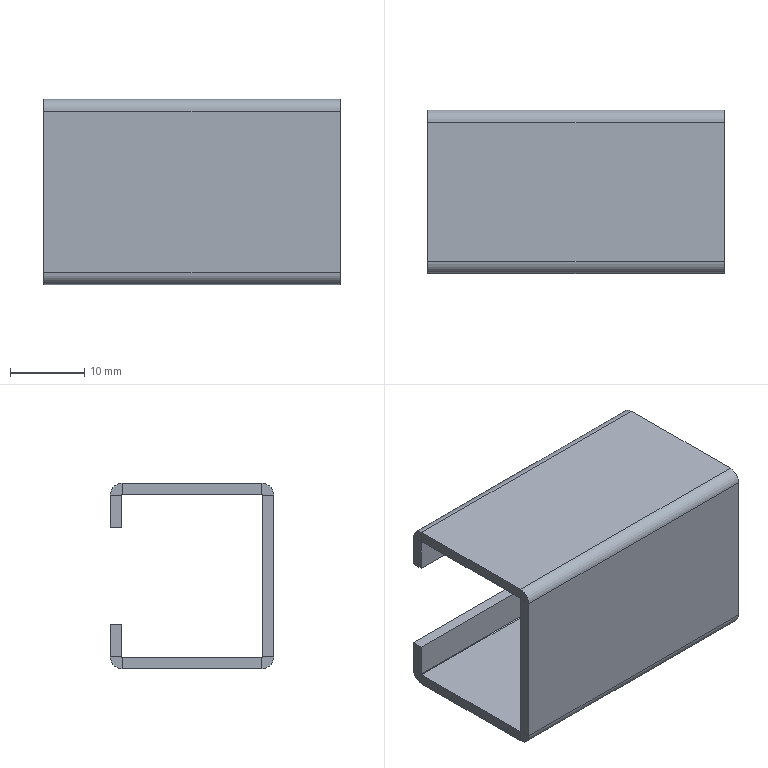Component | SolidWorks | FrontDoorAssembly-1_FrontDoorWelding-1_DoorLockBarGuideSeatPG50-02-106-1 | 1 solid | 38 faces | box 40 x 22 x 25 mm | volume 4412 mm3 | plane 30 | cylinder 8 | commonest cylinder face diameters 3.2 x4 0.2 x4 | material AISI 1045 Steel, cold drawn
STEP:
#1=CARTESIAN_POINT('',(-39.122,-10.291,15.187));
#2=VERTEX_POINT('',#1);
#3=CARTESIAN_POINT('',(-39.122,-10.291,15.246));
#4=VERTEX_POINT('',#3);
#5=CARTESIAN_POINT('',(-39.122,-10.291,15.187));
#6=DIRECTION('',(0.,0.,1.));
#7=VECTOR('',#6,39.37);
#8=LINE('',#5,#7);
#9=EDGE_CURVE('',#2,#4,#8,.T.);
#10=ORIENTED_EDGE('',*,*,#9,.F.);
#11=CARTESIAN_POINT('',(-39.122,-11.031,15.187));
#12=VERTEX_POINT('',#11);
#13=CARTESIAN_POINT('',(-39.122,-11.035,15.187));
#14=DIRECTION('',(0.,-1.,-0.));
#15=VECTOR('',#14,39.37);
#16=LINE('',#13,#15);
#17=EDGE_CURVE('',#2,#12,#16,.T.);
#18=ORIENTED_EDGE('',*,*,#17,.T.);
#19=CARTESIAN_POINT('',(-39.122,-11.031,15.246));
#20=VERTEX_POINT('',#19);
#21=CARTESIAN_POINT('',(-39.122,-11.031,15.246));
#22=DIRECTION('',(0.,-0.,1.));
#23=VECTOR('',#22,39.37);
#24=LINE('',#21,#23);
#25=EDGE_CURVE('',#12,#20,#24,.T.);
#26=ORIENTED_EDGE('',*,*,#25,.T.);
#27=CARTESIAN_POINT('',(-39.122,-11.035,15.246));
#28=DIRECTION('',(0.,-1.,-0.));
#29=VECTOR('',#28,39.37);
#30=LINE('',#27,#29);
#31=EDGE_CURVE('',#4,#20,#30,.T.);
#32=ORIENTED_EDGE('',*,*,#31,.F.);
#33=EDGE_LOOP('',(#10,#18,#26,#32));
#34=FACE_OUTER_BOUND('',#33,.T.);
#35=CARTESIAN_POINT('',(-39.122,-11.035,15.246));
#36=DIRECTION('',(1.,0.,-0.));
#37=DIRECTION('',(-0.,-0.,-1.));
#38=AXIS2_PLACEMENT_3D('',#35,#36,#37);
#39=PLANE('',#38);
#40=ADVANCED_FACE('',(#34),#39,.F.);
#41=CARTESIAN_POINT('',(-37.547,-10.291,15.187));
#42=VERTEX_POINT('',#41);
#43=CARTESIAN_POINT('',(-37.547,-10.291,15.246));
#44=VERTEX_POINT('',#43);
#45=CARTESIAN_POINT('',(-37.547,-10.291,15.187));
#46=DIRECTION('',(0.,0.,1.));
#47=VECTOR('',#46,39.37);
#48=LINE('',#45,#47);
#49=EDGE_CURVE('',#42,#44,#48,.T.);
#50=ORIENTED_EDGE('',*,*,#49,.T.);
#51=CARTESIAN_POINT('',(-37.547,-11.031,15.246));
#52=VERTEX_POINT('',#51);
#53=CARTESIAN_POINT('',(-37.547,-11.035,15.246));
#54=DIRECTION('',(-0.,1.,0.));
#55=VECTOR('',#54,39.37);
#56=LINE('',#53,#55);
#57=EDGE_CURVE('',#52,#44,#56,.T.);
#58=ORIENTED_EDGE('',*,*,#57,.F.);
#59=CARTESIAN_POINT('',(-37.547,-11.031,15.187));
#60=VERTEX_POINT('',#59);
#61=CARTESIAN_POINT('',(-37.547,-11.031,15.187));
#62=DIRECTION('',(0.,-0.,1.));
#63=VECTOR('',#62,39.37);
#64=LINE('',#61,#63);
#65=EDGE_CURVE('',#60,#52,#64,.T.);
#66=ORIENTED_EDGE('',*,*,#65,.F.);
#67=CARTESIAN_POINT('',(-37.547,-10.228,15.187));
#68=DIRECTION('',(-0.,1.,0.));
#69=VECTOR('',#68,39.37);
#70=LINE('',#67,#69);
#71=EDGE_CURVE('',#60,#42,#70,.T.);
#72=ORIENTED_EDGE('',*,*,#71,.T.);
#73=EDGE_LOOP('',(#50,#58,#66,#72));
#74=FACE_OUTER_BOUND('',#73,.T.);
#75=CARTESIAN_POINT('',(-37.547,-10.228,15.246));
#76=DIRECTION('',(-1.,-0.,0.));
#77=DIRECTION('',(0.,0.,1.));
#78=AXIS2_PLACEMENT_3D('',#75,#76,#77);
#79=PLANE('',#78);
#80=ADVANCED_FACE('',(#74),#79,.F.);
#81=CARTESIAN_POINT('',(-37.547,-10.291,15.246));
#82=DIRECTION('',(-1.,-0.,0.));
#83=VECTOR('',#82,39.37);
#84=LINE('',#81,#83);
#85=EDGE_CURVE('',#44,#4,#84,.T.);
#86=ORIENTED_EDGE('',*,*,#85,.T.);
#87=ORIENTED_EDGE('',*,*,#31,.T.);
#88=CARTESIAN_POINT('',(-39.122,-11.031,15.246));
#89=DIRECTION('',(-1.,-0.,0.));
#90=VECTOR('',#89,39.37);
#91=LINE('',#88,#90);
#92=EDGE_CURVE('',#52,#20,#91,.T.);
#93=ORIENTED_EDGE('',*,*,#92,.F.);
#94=ORIENTED_EDGE('',*,*,#57,.T.);
#95=EDGE_LOOP('',(#86,#87,#93,#94));
#96=FACE_OUTER_BOUND('',#95,.T.);
#97=CARTESIAN_POINT('',(-38.334,-11.035,15.246));
#98=DIRECTION('',(-0.,0.,-1.));
#99=DIRECTION('',(-0.,1.,0.));
#100=AXIS2_PLACEMENT_3D('',#97,#98,#99);
#101=PLANE('',#100);
#102=ADVANCED_FACE('',(#96),#101,.F.);
#103=ORIENTED_EDGE('',*,*,#17,.F.);
#104=CARTESIAN_POINT('',(-37.547,-10.291,15.187));
#105=DIRECTION('',(-1.,-0.,0.));
#106=VECTOR('',#105,39.37);
#107=LINE('',#104,#106);
#108=EDGE_CURVE('',#42,#2,#107,.T.);
#109=ORIENTED_EDGE('',*,*,#108,.F.);
#110=ORIENTED_EDGE('',*,*,#71,.F.);
#111=CARTESIAN_POINT('',(-39.122,-11.031,15.187));
#112=DIRECTION('',(1.,0.,-0.));
#113=VECTOR('',#112,39.37);
#114=LINE('',#111,#113);
#115=EDGE_CURVE('',#12,#60,#114,.T.);
#116=ORIENTED_EDGE('',*,*,#115,.F.);
#117=EDGE_LOOP('',(#103,#109,#110,#116));
#118=FACE_OUTER_BOUND('',#117,.T.);
#119=CARTESIAN_POINT('',(-38.334,-11.035,15.187));
#120=DIRECTION('',(-0.,0.,-1.));
#121=DIRECTION('',(-0.,1.,0.));
#122=AXIS2_PLACEMENT_3D('',#119,#120,#121);
#123=PLANE('',#122);
#124=ADVANCED_FACE('',(#118),#123,.T.);
#125=CARTESIAN_POINT('',(-37.547,-10.291,14.321));
#126=VERTEX_POINT('',#125);
#127=CARTESIAN_POINT('',(-37.547,-10.291,14.262));
#128=VERTEX_POINT('',#127);
#129=CARTESIAN_POINT('',(-37.547,-10.291,14.321));
#130=DIRECTION('',(-0.,-0.,-1.));
#131=VECTOR('',#130,39.37);
#132=LINE('',#129,#131);
#133=EDGE_CURVE('',#126,#128,#132,.T.);
#134=ORIENTED_EDGE('',*,*,#133,.F.);
#135=CARTESIAN_POINT('',(-37.547,-11.031,14.321));
#136=VERTEX_POINT('',#135);
#137=CARTESIAN_POINT('',(-37.547,-11.035,14.321));
#138=DIRECTION('',(0.,-1.,0.));
#139=VECTOR('',#138,39.37);
#140=LINE('',#137,#139);
#141=EDGE_CURVE('',#126,#136,#140,.T.);
#142=ORIENTED_EDGE('',*,*,#141,.T.);
#143=CARTESIAN_POINT('',(-37.547,-11.031,14.262));
#144=VERTEX_POINT('',#143);
#145=CARTESIAN_POINT('',(-37.547,-11.031,14.262));
#146=DIRECTION('',(-0.,-0.,-1.));
#147=VECTOR('',#146,39.37);
#148=LINE('',#145,#147);
#149=EDGE_CURVE('',#136,#144,#148,.T.);
#150=ORIENTED_EDGE('',*,*,#149,.T.);
#151=CARTESIAN_POINT('',(-37.547,-11.035,14.262));
#152=DIRECTION('',(0.,-1.,0.));
#153=VECTOR('',#152,39.37);
#154=LINE('',#151,#153);
#155=EDGE_CURVE('',#128,#144,#154,.T.);
#156=ORIENTED_EDGE('',*,*,#155,.F.);
#157=EDGE_LOOP('',(#134,#142,#150,#156));
#158=FACE_OUTER_BOUND('',#157,.T.);
#159=CARTESIAN_POINT('',(-37.547,-11.035,14.262));
#160=DIRECTION('',(-1.,-0.,0.));
#161=DIRECTION('',(-0.,1.,0.));
#162=AXIS2_PLACEMENT_3D('',#159,#160,#161);
#163=PLANE('',#162);
#164=ADVANCED_FACE('',(#158),#163,.F.);
#165=CARTESIAN_POINT('',(-39.122,-10.291,14.321));
#166=VERTEX_POINT('',#165);
#167=CARTESIAN_POINT('',(-39.122,-10.291,14.262));
#168=VERTEX_POINT('',#167);
#169=CARTESIAN_POINT('',(-39.122,-10.291,14.321));
#170=DIRECTION('',(-0.,-0.,-1.));
#171=VECTOR('',#170,39.37);
#172=LINE('',#169,#171);
#173=EDGE_CURVE('',#166,#168,#172,.T.);
#174=ORIENTED_EDGE('',*,*,#173,.T.);
#175=CARTESIAN_POINT('',(-39.122,-11.031,14.262));
#176=VERTEX_POINT('',#175);
#177=CARTESIAN_POINT('',(-39.122,-11.035,14.262));
#178=DIRECTION('',(-0.,1.,-0.));
#179=VECTOR('',#178,39.37);
#180=LINE('',#177,#179);
#181=EDGE_CURVE('',#176,#168,#180,.T.);
#182=ORIENTED_EDGE('',*,*,#181,.F.);
#183=CARTESIAN_POINT('',(-39.122,-11.031,14.321));
#184=VERTEX_POINT('',#183);
#185=CARTESIAN_POINT('',(-39.122,-11.031,14.321));
#186=DIRECTION('',(-0.,-0.,-1.));
#187=VECTOR('',#186,39.37);
#188=LINE('',#185,#187);
#189=EDGE_CURVE('',#184,#176,#188,.T.);
#190=ORIENTED_EDGE('',*,*,#189,.F.);
#191=CARTESIAN_POINT('',(-39.122,-10.228,14.321));
#192=DIRECTION('',(-0.,1.,-0.));
#193=VECTOR('',#192,39.37);
#194=LINE('',#191,#193);
#195=EDGE_CURVE('',#184,#166,#194,.T.);
#196=ORIENTED_EDGE('',*,*,#195,.T.);
#197=EDGE_LOOP('',(#174,#182,#190,#196));
#198=FACE_OUTER_BOUND('',#197,.T.);
#199=CARTESIAN_POINT('',(-39.122,-10.228,14.262));
#200=DIRECTION('',(1.,0.,-0.));
#201=DIRECTION('',(0.,-1.,-0.));
#202=AXIS2_PLACEMENT_3D('',#199,#200,#201);
#203=PLANE('',#202);
#204=ADVANCED_FACE('',(#198),#203,.F.);
#205=CARTESIAN_POINT('',(-39.122,-10.291,14.262));
#206=DIRECTION('',(1.,0.,-0.));
#207=VECTOR('',#206,39.37);
#208=LINE('',#205,#207);
#209=EDGE_CURVE('',#168,#128,#208,.T.);
#210=ORIENTED_EDGE('',*,*,#209,.T.);
#211=ORIENTED_EDGE('',*,*,#155,.T.);
#212=CARTESIAN_POINT('',(-37.547,-11.031,14.262));
#213=DIRECTION('',(1.,0.,-0.));
#214=VECTOR('',#213,39.37);
#215=LINE('',#212,#214);
#216=EDGE_CURVE('',#176,#144,#215,.T.);
#217=ORIENTED_EDGE('',*,*,#216,.F.);
#218=ORIENTED_EDGE('',*,*,#181,.T.);
#219=EDGE_LOOP('',(#210,#211,#217,#218));
#220=FACE_OUTER_BOUND('',#219,.T.);
#221=CARTESIAN_POINT('',(-38.334,-11.035,14.262));
#222=DIRECTION('',(0.,0.,1.));
#223=DIRECTION('',(0.,-1.,0.));
#224=AXIS2_PLACEMENT_3D('',#221,#222,#223);
#225=PLANE('',#224);
#226=ADVANCED_FACE('',(#220),#225,.F.);
#227=ORIENTED_EDGE('',*,*,#141,.F.);
#228=CARTESIAN_POINT('',(-39.122,-10.291,14.321));
#229=DIRECTION('',(1.,0.,-0.));
#230=VECTOR('',#229,39.37);
#231=LINE('',#228,#230);
#232=EDGE_CURVE('',#166,#126,#231,.T.);
#233=ORIENTED_EDGE('',*,*,#232,.F.);
#234=ORIENTED_EDGE('',*,*,#195,.F.);
#235=CARTESIAN_POINT('',(-37.547,-11.031,14.321));
#236=DIRECTION('',(-1.,-0.,0.));
#237=VECTOR('',#236,39.37);
#238=LINE('',#235,#237);
#239=EDGE_CURVE('',#136,#184,#238,.T.);
#240=ORIENTED_EDGE('',*,*,#239,.F.);
#241=EDGE_LOOP('',(#227,#233,#234,#240));
#242=FACE_OUTER_BOUND('',#241,.T.);
#243=CARTESIAN_POINT('',(-38.334,-11.035,14.321));
#244=DIRECTION('',(0.,0.,1.));
#245=DIRECTION('',(0.,-1.,0.));
#246=AXIS2_PLACEMENT_3D('',#243,#244,#245);
#247=PLANE('',#246);
#248=ADVANCED_FACE('',(#242),#247,.T.);
#249=CARTESIAN_POINT('',(-37.547,-11.094,15.183));
#250=VERTEX_POINT('',#249);
#251=CARTESIAN_POINT('',(-37.547,-11.094,14.325));
#252=VERTEX_POINT('',#251);
#253=CARTESIAN_POINT('',(-37.547,-11.094,14.262));
#254=DIRECTION('',(-0.,-0.,-1.));
#255=VECTOR('',#254,39.37);
#256=LINE('',#253,#255);
#257=EDGE_CURVE('',#250,#252,#256,.T.);
#258=ORIENTED_EDGE('',*,*,#257,.F.);
#259=CARTESIAN_POINT('',(-39.122,-11.094,15.183));
#260=VERTEX_POINT('',#259);
#261=CARTESIAN_POINT('',(-37.547,-11.094,15.183));
#262=DIRECTION('',(-1.,-0.,0.));
#263=VECTOR('',#262,39.37);
#264=LINE('',#261,#263);
#265=EDGE_CURVE('',#250,#260,#264,.T.);
#266=ORIENTED_EDGE('',*,*,#265,.T.);
#267=CARTESIAN_POINT('',(-39.122,-11.094,14.325));
#268=VERTEX_POINT('',#267);
#269=CARTESIAN_POINT('',(-39.122,-11.094,14.262));
#270=DIRECTION('',(0.,0.,1.));
#271=VECTOR('',#270,39.37);
#272=LINE('',#269,#271);
#273=EDGE_CURVE('',#268,#260,#272,.T.);
#274=ORIENTED_EDGE('',*,*,#273,.F.);
#275=CARTESIAN_POINT('',(-39.122,-11.094,14.325));
#276=DIRECTION('',(1.,0.,-0.));
#277=VECTOR('',#276,39.37);
#278=LINE('',#275,#277);
#279=EDGE_CURVE('',#268,#252,#278,.T.);
#280=ORIENTED_EDGE('',*,*,#279,.T.);
#281=EDGE_LOOP('',(#258,#266,#274,#280));
#282=FACE_OUTER_BOUND('',#281,.T.);
#283=CARTESIAN_POINT('',(-38.334,-11.094,14.754));
#284=DIRECTION('',(0.,-1.,-0.));
#285=DIRECTION('',(-1.,-0.,0.));
#286=AXIS2_PLACEMENT_3D('',#283,#284,#285);
#287=PLANE('',#286);
#288=ADVANCED_FACE('',(#282),#287,.T.);
#289=CARTESIAN_POINT('',(-37.547,-11.035,15.183));
#290=VERTEX_POINT('',#289);
#291=CARTESIAN_POINT('',(-39.122,-11.035,15.183));
#292=VERTEX_POINT('',#291);
#293=CARTESIAN_POINT('',(-37.547,-11.035,15.183));
#294=DIRECTION('',(-1.,-0.,0.));
#295=VECTOR('',#294,39.37);
#296=LINE('',#293,#295);
#297=EDGE_CURVE('',#290,#292,#296,.T.);
#298=ORIENTED_EDGE('',*,*,#297,.F.);
#299=CARTESIAN_POINT('',(-37.547,-11.035,14.325));
#300=VERTEX_POINT('',#299);
#301=CARTESIAN_POINT('',(-37.547,-11.035,14.262));
#302=DIRECTION('',(-0.,-0.,-1.));
#303=VECTOR('',#302,39.37);
#304=LINE('',#301,#303);
#305=EDGE_CURVE('',#290,#300,#304,.T.);
#306=ORIENTED_EDGE('',*,*,#305,.T.);
#307=CARTESIAN_POINT('',(-39.122,-11.035,14.325));
#308=VERTEX_POINT('',#307);
#309=CARTESIAN_POINT('',(-39.122,-11.035,14.325));
#310=DIRECTION('',(1.,0.,-0.));
#311=VECTOR('',#310,39.37);
#312=LINE('',#309,#311);
#313=EDGE_CURVE('',#308,#300,#312,.T.);
#314=ORIENTED_EDGE('',*,*,#313,.F.);
#315=CARTESIAN_POINT('',(-39.122,-11.035,14.262));
#316=DIRECTION('',(0.,0.,1.));
#317=VECTOR('',#316,39.37);
#318=LINE('',#315,#317);
#319=EDGE_CURVE('',#308,#292,#318,.T.);
#320=ORIENTED_EDGE('',*,*,#319,.T.);
#321=EDGE_LOOP('',(#298,#306,#314,#320));
#322=FACE_OUTER_BOUND('',#321,.T.);
#323=CARTESIAN_POINT('',(-38.334,-11.035,14.754));
#324=DIRECTION('',(0.,-1.,-0.));
#325=DIRECTION('',(-1.,-0.,0.));
#326=AXIS2_PLACEMENT_3D('',#323,#324,#325);
#327=PLANE('',#326);
#328=ADVANCED_FACE('',(#322),#327,.F.);
#329=ORIENTED_EDGE('',*,*,#305,.F.);
#330=CARTESIAN_POINT('',(-37.547,-11.035,15.183));
#331=DIRECTION('',(0.,-1.,-0.));
#332=VECTOR('',#331,39.37);
#333=LINE('',#330,#332);
#334=EDGE_CURVE('',#290,#250,#333,.T.);
#335=ORIENTED_EDGE('',*,*,#334,.T.);
#336=ORIENTED_EDGE('',*,*,#257,.T.);
#337=CARTESIAN_POINT('',(-37.547,-11.035,14.325));
#338=DIRECTION('',(0.,-1.,0.));
#339=VECTOR('',#338,39.37);
#340=LINE('',#337,#339);
#341=EDGE_CURVE('',#300,#252,#340,.T.);
#342=ORIENTED_EDGE('',*,*,#341,.F.);
#343=EDGE_LOOP('',(#329,#335,#336,#342));
#344=FACE_OUTER_BOUND('',#343,.T.);
#345=CARTESIAN_POINT('',(-37.547,-11.094,14.262));
#346=DIRECTION('',(1.,0.,-0.));
#347=DIRECTION('',(-0.,-0.,-1.));
#348=AXIS2_PLACEMENT_3D('',#345,#346,#347);
#349=PLANE('',#348);
#350=ADVANCED_FACE('',(#344),#349,.T.);
#351=CARTESIAN_POINT('',(-39.122,-11.035,15.183));
#352=DIRECTION('',(0.,-1.,-0.));
#353=VECTOR('',#352,39.37);
#354=LINE('',#351,#353);
#355=EDGE_CURVE('',#292,#260,#354,.T.);
#356=ORIENTED_EDGE('',*,*,#355,.F.);
#357=ORIENTED_EDGE('',*,*,#319,.F.);
#358=CARTESIAN_POINT('',(-39.122,-11.035,14.325));
#359=DIRECTION('',(0.,-1.,0.));
#360=VECTOR('',#359,39.37);
#361=LINE('',#358,#360);
#362=EDGE_CURVE('',#308,#268,#361,.T.);
#363=ORIENTED_EDGE('',*,*,#362,.T.);
#364=ORIENTED_EDGE('',*,*,#273,.T.);
#365=EDGE_LOOP('',(#356,#357,#363,#364));
#366=FACE_OUTER_BOUND('',#365,.T.);
#367=CARTESIAN_POINT('',(-39.122,-11.094,14.262));
#368=DIRECTION('',(-1.,-0.,0.));
#369=DIRECTION('',(0.,0.,1.));
#370=AXIS2_PLACEMENT_3D('',#367,#368,#369);
#371=PLANE('',#370);
#372=ADVANCED_FACE('',(#366),#371,.T.);
#373=ORIENTED_EDGE('',*,*,#149,.F.);
#374=CARTESIAN_POINT('',(-37.547,-11.031,14.325));
#375=DIRECTION('',(1.,0.,-0.));
#376=DIRECTION('',(0.,1.,0.));
#377=AXIS2_PLACEMENT_3D('',#374,#375,#376);
#378=CIRCLE('',#377,0.003937);
#379=EDGE_CURVE('',#300,#136,#378,.T.);
#380=ORIENTED_EDGE('',*,*,#379,.F.);
#381=ORIENTED_EDGE('',*,*,#341,.T.);
#382=CARTESIAN_POINT('',(-37.547,-11.031,14.325));
#383=DIRECTION('',(1.,0.,-0.));
#384=DIRECTION('',(0.,1.,0.));
#385=AXIS2_PLACEMENT_3D('',#382,#383,#384);
#386=CIRCLE('',#385,0.06299);
#387=EDGE_CURVE('',#252,#144,#386,.T.);
#388=ORIENTED_EDGE('',*,*,#387,.T.);
#389=EDGE_LOOP('',(#373,#380,#381,#388));
#390=FACE_OUTER_BOUND('',#389,.T.);
#391=CARTESIAN_POINT('',(-37.547,-11.031,14.325));
#392=DIRECTION('',(1.,0.,-0.));
#393=DIRECTION('',(0.,-1.,-0.));
#394=AXIS2_PLACEMENT_3D('',#391,#392,#393);
#395=PLANE('',#394);
#396=ADVANCED_FACE('',(#390),#395,.T.);
#397=CARTESIAN_POINT('',(-39.122,-11.031,14.325));
#398=DIRECTION('',(-1.,-0.,0.));
#399=DIRECTION('',(0.,1.,0.));
#400=AXIS2_PLACEMENT_3D('',#397,#398,#399);
#401=CIRCLE('',#400,0.003937);
#402=EDGE_CURVE('',#184,#308,#401,.T.);
#403=ORIENTED_EDGE('',*,*,#402,.F.);
#404=ORIENTED_EDGE('',*,*,#189,.T.);
#405=CARTESIAN_POINT('',(-39.122,-11.031,14.325));
#406=DIRECTION('',(-1.,-0.,0.));
#407=DIRECTION('',(0.,1.,0.));
#408=AXIS2_PLACEMENT_3D('',#405,#406,#407);
#409=CIRCLE('',#408,0.06299);
#410=EDGE_CURVE('',#176,#268,#409,.T.);
#411=ORIENTED_EDGE('',*,*,#410,.T.);
#412=ORIENTED_EDGE('',*,*,#362,.F.);
#413=EDGE_LOOP('',(#403,#404,#411,#412));
#414=FACE_OUTER_BOUND('',#413,.T.);
#415=CARTESIAN_POINT('',(-39.122,-11.031,14.325));
#416=DIRECTION('',(1.,0.,-0.));
#417=DIRECTION('',(0.,-1.,-0.));
#418=AXIS2_PLACEMENT_3D('',#415,#416,#417);
#419=PLANE('',#418);
#420=ADVANCED_FACE('',(#414),#419,.F.);
#421=ORIENTED_EDGE('',*,*,#279,.F.);
#422=ORIENTED_EDGE('',*,*,#410,.F.);
#423=ORIENTED_EDGE('',*,*,#216,.T.);
#424=ORIENTED_EDGE('',*,*,#387,.F.);
#425=EDGE_LOOP('',(#421,#422,#423,#424));
#426=FACE_OUTER_BOUND('',#425,.T.);
#427=CARTESIAN_POINT('',(-39.122,-11.031,14.325));
#428=DIRECTION('',(-1.,-0.,0.));
#429=DIRECTION('',(0.,0.,-1.));
#430=AXIS2_PLACEMENT_3D('',#427,#428,#429);
#431=CYLINDRICAL_SURFACE('',#430,0.06299);
#432=ADVANCED_FACE('',(#426),#431,.T.);
#433=ORIENTED_EDGE('',*,*,#313,.T.);
#434=ORIENTED_EDGE('',*,*,#379,.T.);
#435=ORIENTED_EDGE('',*,*,#239,.T.);
#436=ORIENTED_EDGE('',*,*,#402,.T.);
#437=EDGE_LOOP('',(#433,#434,#435,#436));
#438=FACE_OUTER_BOUND('',#437,.T.);
#439=CARTESIAN_POINT('',(-39.122,-11.031,14.325));
#440=DIRECTION('',(-1.,-0.,0.));
#441=DIRECTION('',(0.,0.,-1.));
#442=AXIS2_PLACEMENT_3D('',#439,#440,#441);
#443=CYLINDRICAL_SURFACE('',#442,0.003937);
#444=ADVANCED_FACE('',(#438),#443,.F.);
#445=ORIENTED_EDGE('',*,*,#25,.F.);
#446=CARTESIAN_POINT('',(-39.122,-11.031,15.183));
#447=DIRECTION('',(-1.,-0.,0.));
#448=DIRECTION('',(0.,-1.,0.));
#449=AXIS2_PLACEMENT_3D('',#446,#447,#448);
#450=CIRCLE('',#449,0.003937);
#451=EDGE_CURVE('',#292,#12,#450,.T.);
#452=ORIENTED_EDGE('',*,*,#451,.F.);
#453=ORIENTED_EDGE('',*,*,#355,.T.);
#454=CARTESIAN_POINT('',(-39.122,-11.031,15.183));
#455=DIRECTION('',(-1.,-0.,0.));
#456=DIRECTION('',(0.,-1.,0.));
#457=AXIS2_PLACEMENT_3D('',#454,#455,#456);
#458=CIRCLE('',#457,0.06299);
#459=EDGE_CURVE('',#260,#20,#458,.T.);
#460=ORIENTED_EDGE('',*,*,#459,.T.);
#461=EDGE_LOOP('',(#445,#452,#453,#460));
#462=FACE_OUTER_BOUND('',#461,.T.);
#463=CARTESIAN_POINT('',(-39.122,-11.031,15.183));
#464=DIRECTION('',(-1.,-0.,0.));
#465=DIRECTION('',(-0.,1.,0.));
#466=AXIS2_PLACEMENT_3D('',#463,#464,#465);
#467=PLANE('',#466);
#468=ADVANCED_FACE('',(#462),#467,.T.);
#469=CARTESIAN_POINT('',(-37.547,-11.031,15.183));
#470=DIRECTION('',(1.,0.,-0.));
#471=DIRECTION('',(0.,-1.,0.));
#472=AXIS2_PLACEMENT_3D('',#469,#470,#471);
#473=CIRCLE('',#472,0.003937);
#474=EDGE_CURVE('',#60,#290,#473,.T.);
#475=ORIENTED_EDGE('',*,*,#474,.F.);
#476=ORIENTED_EDGE('',*,*,#65,.T.);
#477=CARTESIAN_POINT('',(-37.547,-11.031,15.183));
#478=DIRECTION('',(1.,0.,-0.));
#479=DIRECTION('',(0.,-1.,0.));
#480=AXIS2_PLACEMENT_3D('',#477,#478,#479);
#481=CIRCLE('',#480,0.06299);
#482=EDGE_CURVE('',#52,#250,#481,.T.);
#483=ORIENTED_EDGE('',*,*,#482,.T.);
#484=ORIENTED_EDGE('',*,*,#334,.F.);
#485=EDGE_LOOP('',(#475,#476,#483,#484));
#486=FACE_OUTER_BOUND('',#485,.T.);
#487=CARTESIAN_POINT('',(-37.547,-11.031,15.183));
#488=DIRECTION('',(-1.,-0.,0.));
#489=DIRECTION('',(-0.,1.,0.));
#490=AXIS2_PLACEMENT_3D('',#487,#488,#489);
#491=PLANE('',#490);
#492=ADVANCED_FACE('',(#486),#491,.F.);
#493=ORIENTED_EDGE('',*,*,#265,.F.);
#494=ORIENTED_EDGE('',*,*,#482,.F.);
#495=ORIENTED_EDGE('',*,*,#92,.T.);
#496=ORIENTED_EDGE('',*,*,#459,.F.);
#497=EDGE_LOOP('',(#493,#494,#495,#496));
#498=FACE_OUTER_BOUND('',#497,.T.);
#499=CARTESIAN_POINT('',(-37.547,-11.031,15.183));
#500=DIRECTION('',(1.,0.,-0.));
#501=DIRECTION('',(0.,0.,1.));
#502=AXIS2_PLACEMENT_3D('',#499,#500,#501);
#503=CYLINDRICAL_SURFACE('',#502,0.06299);
#504=ADVANCED_FACE('',(#498),#503,.T.);
#505=ORIENTED_EDGE('',*,*,#297,.T.);
#506=ORIENTED_EDGE('',*,*,#451,.T.);
#507=ORIENTED_EDGE('',*,*,#115,.T.);
#508=ORIENTED_EDGE('',*,*,#474,.T.);
#509=EDGE_LOOP('',(#505,#506,#507,#508));
#510=FACE_OUTER_BOUND('',#509,.T.);
#511=CARTESIAN_POINT('',(-37.547,-11.031,15.183));
#512=DIRECTION('',(1.,0.,-0.));
#513=DIRECTION('',(0.,0.,1.));
#514=AXIS2_PLACEMENT_3D('',#511,#512,#513);
#515=CYLINDRICAL_SURFACE('',#514,0.003937);
#516=ADVANCED_FACE('',(#510),#515,.F.);
#517=CARTESIAN_POINT('',(-37.547,-10.287,14.325));
#518=VERTEX_POINT('',#517);
#519=CARTESIAN_POINT('',(-37.547,-10.228,14.325));
#520=VERTEX_POINT('',#519);
#521=CARTESIAN_POINT('',(-37.547,-10.228,14.325));
#522=DIRECTION('',(-0.,1.,0.));
#523=VECTOR('',#522,39.37);
#524=LINE('',#521,#523);
#525=EDGE_CURVE('',#518,#520,#524,.T.);
#526=ORIENTED_EDGE('',*,*,#525,.F.);
#527=CARTESIAN_POINT('',(-37.547,-10.291,14.325));
#528=DIRECTION('',(1.,0.,-0.));
#529=DIRECTION('',(0.,1.,0.));
#530=AXIS2_PLACEMENT_3D('',#527,#528,#529);
#531=CIRCLE('',#530,0.003937);
#532=EDGE_CURVE('',#126,#518,#531,.T.);
#533=ORIENTED_EDGE('',*,*,#532,.F.);
#534=ORIENTED_EDGE('',*,*,#133,.T.);
#535=CARTESIAN_POINT('',(-37.547,-10.291,14.325));
#536=DIRECTION('',(1.,0.,-0.));
#537=DIRECTION('',(0.,1.,0.));
#538=AXIS2_PLACEMENT_3D('',#535,#536,#537);
#539=CIRCLE('',#538,0.06299);
#540=EDGE_CURVE('',#128,#520,#539,.T.);
#541=ORIENTED_EDGE('',*,*,#540,.T.);
#542=EDGE_LOOP('',(#526,#533,#534,#541));
#543=FACE_OUTER_BOUND('',#542,.T.);
#544=CARTESIAN_POINT('',(-37.547,-10.291,14.325));
#545=DIRECTION('',(1.,0.,-0.));
#546=DIRECTION('',(0.,-1.,-0.));
#547=AXIS2_PLACEMENT_3D('',#544,#545,#546);
#548=PLANE('',#547);
#549=ADVANCED_FACE('',(#543),#548,.T.);
#550=CARTESIAN_POINT('',(-39.122,-10.287,14.325));
#551=VERTEX_POINT('',#550);
#552=CARTESIAN_POINT('',(-39.122,-10.291,14.325));
#553=DIRECTION('',(-1.,-0.,0.));
#554=DIRECTION('',(0.,1.,0.));
#555=AXIS2_PLACEMENT_3D('',#552,#553,#554);
#556=CIRCLE('',#555,0.003937);
#557=EDGE_CURVE('',#551,#166,#556,.T.);
#558=ORIENTED_EDGE('',*,*,#557,.F.);
#559=CARTESIAN_POINT('',(-39.122,-10.228,14.325));
#560=VERTEX_POINT('',#559);
#561=CARTESIAN_POINT('',(-39.122,-10.287,14.325));
#562=DIRECTION('',(-0.,1.,0.));
#563=VECTOR('',#562,39.37);
#564=LINE('',#561,#563);
#565=EDGE_CURVE('',#551,#560,#564,.T.);
#566=ORIENTED_EDGE('',*,*,#565,.T.);
#567=CARTESIAN_POINT('',(-39.122,-10.291,14.325));
#568=DIRECTION('',(-1.,-0.,0.));
#569=DIRECTION('',(0.,1.,0.));
#570=AXIS2_PLACEMENT_3D('',#567,#568,#569);
#571=CIRCLE('',#570,0.06299);
#572=EDGE_CURVE('',#560,#168,#571,.T.);
#573=ORIENTED_EDGE('',*,*,#572,.T.);
#574=ORIENTED_EDGE('',*,*,#173,.F.);
#575=EDGE_LOOP('',(#558,#566,#573,#574));
#576=FACE_OUTER_BOUND('',#575,.T.);
#577=CARTESIAN_POINT('',(-39.122,-10.291,14.325));
#578=DIRECTION('',(1.,0.,-0.));
#579=DIRECTION('',(0.,-1.,-0.));
#580=AXIS2_PLACEMENT_3D('',#577,#578,#579);
#581=PLANE('',#580);
#582=ADVANCED_FACE('',(#576),#581,.F.);
#583=ORIENTED_EDGE('',*,*,#209,.F.);
#584=ORIENTED_EDGE('',*,*,#572,.F.);
#585=CARTESIAN_POINT('',(-37.547,-10.228,14.325));
#586=DIRECTION('',(1.,0.,-0.));
#587=VECTOR('',#586,39.37);
#588=LINE('',#585,#587);
#589=EDGE_CURVE('',#560,#520,#588,.T.);
#590=ORIENTED_EDGE('',*,*,#589,.T.);
#591=ORIENTED_EDGE('',*,*,#540,.F.);
#592=EDGE_LOOP('',(#583,#584,#590,#591));
#593=FACE_OUTER_BOUND('',#592,.T.);
#594=CARTESIAN_POINT('',(-39.122,-10.291,14.325));
#595=DIRECTION('',(-1.,-0.,0.));
#596=DIRECTION('',(0.,1.,0.));
#597=AXIS2_PLACEMENT_3D('',#594,#595,#596);
#598=CYLINDRICAL_SURFACE('',#597,0.06299);
#599=ADVANCED_FACE('',(#593),#598,.T.);
#600=ORIENTED_EDGE('',*,*,#232,.T.);
#601=ORIENTED_EDGE('',*,*,#532,.T.);
#602=CARTESIAN_POINT('',(-37.547,-10.287,14.325));
#603=DIRECTION('',(-1.,-0.,0.));
#604=VECTOR('',#603,39.37);
#605=LINE('',#602,#604);
#606=EDGE_CURVE('',#518,#551,#605,.T.);
#607=ORIENTED_EDGE('',*,*,#606,.T.);
#608=ORIENTED_EDGE('',*,*,#557,.T.);
#609=EDGE_LOOP('',(#600,#601,#607,#608));
#610=FACE_OUTER_BOUND('',#609,.T.);
#611=CARTESIAN_POINT('',(-39.122,-10.291,14.325));
#612=DIRECTION('',(-1.,-0.,0.));
#613=DIRECTION('',(0.,1.,0.));
#614=AXIS2_PLACEMENT_3D('',#611,#612,#613);
#615=CYLINDRICAL_SURFACE('',#614,0.003937);
#616=ADVANCED_FACE('',(#610),#615,.F.);
#617=ORIENTED_EDGE('',*,*,#565,.F.);
#618=CARTESIAN_POINT('',(-39.122,-10.287,14.498));
#619=VERTEX_POINT('',#618);
#620=CARTESIAN_POINT('',(-39.122,-10.287,14.498));
#621=DIRECTION('',(0.,0.,1.));
#622=VECTOR('',#621,39.37);
#623=LINE('',#620,#622);
#624=EDGE_CURVE('',#551,#619,#623,.T.);
#625=ORIENTED_EDGE('',*,*,#624,.T.);
#626=CARTESIAN_POINT('',(-39.122,-10.228,14.498));
#627=VERTEX_POINT('',#626);
#628=CARTESIAN_POINT('',(-39.122,-10.228,14.498));
#629=DIRECTION('',(0.,-1.,0.));
#630=VECTOR('',#629,39.37);
#631=LINE('',#628,#630);
#632=EDGE_CURVE('',#627,#619,#631,.T.);
#633=ORIENTED_EDGE('',*,*,#632,.F.);
#634=CARTESIAN_POINT('',(-39.122,-10.228,14.754));
#635=DIRECTION('',(0.,0.,1.));
#636=VECTOR('',#635,39.37);
#637=LINE('',#634,#636);
#638=EDGE_CURVE('',#560,#627,#637,.T.);
#639=ORIENTED_EDGE('',*,*,#638,.F.);
#640=EDGE_LOOP('',(#617,#625,#633,#639));
#641=FACE_OUTER_BOUND('',#640,.T.);
#642=CARTESIAN_POINT('',(-39.122,-10.228,14.498));
#643=DIRECTION('',(1.,0.,-0.));
#644=DIRECTION('',(0.,-1.,-0.));
#645=AXIS2_PLACEMENT_3D('',#642,#643,#644);
#646=PLANE('',#645);
#647=ADVANCED_FACE('',(#641),#646,.F.);
#648=ORIENTED_EDGE('',*,*,#525,.T.);
#649=CARTESIAN_POINT('',(-37.547,-10.228,14.498));
#650=VERTEX_POINT('',#649);
#651=CARTESIAN_POINT('',(-37.547,-10.228,14.754));
#652=DIRECTION('',(-0.,-0.,-1.));
#653=VECTOR('',#652,39.37);
#654=LINE('',#651,#653);
#655=EDGE_CURVE('',#650,#520,#654,.T.);
#656=ORIENTED_EDGE('',*,*,#655,.F.);
#657=CARTESIAN_POINT('',(-37.547,-10.287,14.498));
#658=VERTEX_POINT('',#657);
#659=CARTESIAN_POINT('',(-37.547,-10.228,14.498));
#660=DIRECTION('',(0.,-1.,0.));
#661=VECTOR('',#660,39.37);
#662=LINE('',#659,#661);
#663=EDGE_CURVE('',#650,#658,#662,.T.);
#664=ORIENTED_EDGE('',*,*,#663,.T.);
#665=CARTESIAN_POINT('',(-37.547,-10.287,14.321));
#666=DIRECTION('',(-0.,-0.,-1.));
#667=VECTOR('',#666,39.37);
#668=LINE('',#665,#667);
#669=EDGE_CURVE('',#658,#518,#668,.T.);
#670=ORIENTED_EDGE('',*,*,#669,.T.);
#671=EDGE_LOOP('',(#648,#656,#664,#670));
#672=FACE_OUTER_BOUND('',#671,.T.);
#673=CARTESIAN_POINT('',(-37.547,-10.228,14.321));
#674=DIRECTION('',(-1.,-0.,0.));
#675=DIRECTION('',(-0.,1.,0.));
#676=AXIS2_PLACEMENT_3D('',#673,#674,#675);
#677=PLANE('',#676);
#678=ADVANCED_FACE('',(#672),#677,.F.);
#679=ORIENTED_EDGE('',*,*,#589,.F.);
#680=ORIENTED_EDGE('',*,*,#638,.T.);
#681=CARTESIAN_POINT('',(-38.334,-10.228,14.498));
#682=DIRECTION('',(1.,0.,-0.));
#683=VECTOR('',#682,39.37);
#684=LINE('',#681,#683);
#685=EDGE_CURVE('',#627,#650,#684,.T.);
#686=ORIENTED_EDGE('',*,*,#685,.T.);
#687=ORIENTED_EDGE('',*,*,#655,.T.);
#688=EDGE_LOOP('',(#679,#680,#686,#687));
#689=FACE_OUTER_BOUND('',#688,.T.);
#690=CARTESIAN_POINT('',(-38.334,-10.228,14.754));
#691=DIRECTION('',(0.,-1.,0.));
#692=DIRECTION('',(-0.,-0.,-1.));
#693=AXIS2_PLACEMENT_3D('',#690,#691,#692);
#694=PLANE('',#693);
#695=ADVANCED_FACE('',(#689),#694,.F.);
#696=ORIENTED_EDGE('',*,*,#624,.F.);
#697=ORIENTED_EDGE('',*,*,#606,.F.);
#698=ORIENTED_EDGE('',*,*,#669,.F.);
#699=CARTESIAN_POINT('',(-37.547,-10.287,14.498));
#700=DIRECTION('',(1.,0.,-0.));
#701=VECTOR('',#700,39.37);
#702=LINE('',#699,#701);
#703=EDGE_CURVE('',#619,#658,#702,.T.);
#704=ORIENTED_EDGE('',*,*,#703,.F.);
#705=EDGE_LOOP('',(#696,#697,#698,#704));
#706=FACE_OUTER_BOUND('',#705,.T.);
#707=CARTESIAN_POINT('',(-38.334,-10.287,14.754));
#708=DIRECTION('',(0.,-1.,0.));
#709=DIRECTION('',(-0.,-0.,-1.));
#710=AXIS2_PLACEMENT_3D('',#707,#708,#709);
#711=PLANE('',#710);
#712=ADVANCED_FACE('',(#706),#711,.T.);
#713=ORIENTED_EDGE('',*,*,#703,.T.);
#714=ORIENTED_EDGE('',*,*,#663,.F.);
#715=ORIENTED_EDGE('',*,*,#685,.F.);
#716=ORIENTED_EDGE('',*,*,#632,.T.);
#717=EDGE_LOOP('',(#713,#714,#715,#716));
#718=FACE_OUTER_BOUND('',#717,.T.);
#719=CARTESIAN_POINT('',(-37.547,-10.228,14.498));
#720=DIRECTION('',(-0.,-0.,-1.));
#721=DIRECTION('',(-0.,1.,-0.));
#722=AXIS2_PLACEMENT_3D('',#719,#720,#721);
#723=PLANE('',#722);
#724=ADVANCED_FACE('',(#718),#723,.F.);
#725=CARTESIAN_POINT('',(-39.122,-10.287,15.183));
#726=VERTEX_POINT('',#725);
#727=CARTESIAN_POINT('',(-39.122,-10.228,15.183));
#728=VERTEX_POINT('',#727);
#729=CARTESIAN_POINT('',(-39.122,-10.228,15.183));
#730=DIRECTION('',(-0.,1.,0.));
#731=VECTOR('',#730,39.37);
#732=LINE('',#729,#731);
#733=EDGE_CURVE('',#726,#728,#732,.T.);
#734=ORIENTED_EDGE('',*,*,#733,.F.);
#735=CARTESIAN_POINT('',(-39.122,-10.291,15.183));
#736=DIRECTION('',(-1.,-0.,0.));
#737=DIRECTION('',(0.,-1.,0.));
#738=AXIS2_PLACEMENT_3D('',#735,#736,#737);
#739=CIRCLE('',#738,0.003937);
#740=EDGE_CURVE('',#2,#726,#739,.T.);
#741=ORIENTED_EDGE('',*,*,#740,.F.);
#742=ORIENTED_EDGE('',*,*,#9,.T.);
#743=CARTESIAN_POINT('',(-39.122,-10.291,15.183));
#744=DIRECTION('',(-1.,-0.,0.));
#745=DIRECTION('',(0.,-1.,0.));
#746=AXIS2_PLACEMENT_3D('',#743,#744,#745);
#747=CIRCLE('',#746,0.06299);
#748=EDGE_CURVE('',#4,#728,#747,.T.);
#749=ORIENTED_EDGE('',*,*,#748,.T.);
#750=EDGE_LOOP('',(#734,#741,#742,#749));
#751=FACE_OUTER_BOUND('',#750,.T.);
#752=CARTESIAN_POINT('',(-39.122,-10.291,15.183));
#753=DIRECTION('',(-1.,-0.,0.));
#754=DIRECTION('',(-0.,1.,0.));
#755=AXIS2_PLACEMENT_3D('',#752,#753,#754);
#756=PLANE('',#755);
#757=ADVANCED_FACE('',(#751),#756,.T.);
#758=CARTESIAN_POINT('',(-37.547,-10.287,15.183));
#759=VERTEX_POINT('',#758);
#760=CARTESIAN_POINT('',(-37.547,-10.291,15.183));
#761=DIRECTION('',(1.,0.,-0.));
#762=DIRECTION('',(0.,-1.,0.));
#763=AXIS2_PLACEMENT_3D('',#760,#761,#762);
#764=CIRCLE('',#763,0.003937);
#765=EDGE_CURVE('',#759,#42,#764,.T.);
#766=ORIENTED_EDGE('',*,*,#765,.F.);
#767=CARTESIAN_POINT('',(-37.547,-10.228,15.183));
#768=VERTEX_POINT('',#767);
#769=CARTESIAN_POINT('',(-37.547,-10.287,15.183));
#770=DIRECTION('',(-0.,1.,0.));
#771=VECTOR('',#770,39.37);
#772=LINE('',#769,#771);
#773=EDGE_CURVE('',#759,#768,#772,.T.);
#774=ORIENTED_EDGE('',*,*,#773,.T.);
#775=CARTESIAN_POINT('',(-37.547,-10.291,15.183));
#776=DIRECTION('',(1.,0.,-0.));
#777=DIRECTION('',(0.,-1.,0.));
#778=AXIS2_PLACEMENT_3D('',#775,#776,#777);
#779=CIRCLE('',#778,0.06299);
#780=EDGE_CURVE('',#768,#44,#779,.T.);
#781=ORIENTED_EDGE('',*,*,#780,.T.);
#782=ORIENTED_EDGE('',*,*,#49,.F.);
#783=EDGE_LOOP('',(#766,#774,#781,#782));
#784=FACE_OUTER_BOUND('',#783,.T.);
#785=CARTESIAN_POINT('',(-37.547,-10.291,15.183));
#786=DIRECTION('',(-1.,-0.,0.));
#787=DIRECTION('',(-0.,1.,0.));
#788=AXIS2_PLACEMENT_3D('',#785,#786,#787);
#789=PLANE('',#788);
#790=ADVANCED_FACE('',(#784),#789,.F.);
#791=ORIENTED_EDGE('',*,*,#85,.F.);
#792=ORIENTED_EDGE('',*,*,#780,.F.);
#793=CARTESIAN_POINT('',(-39.122,-10.228,15.183));
#794=DIRECTION('',(-1.,-0.,0.));
#795=VECTOR('',#794,39.37);
#796=LINE('',#793,#795);
#797=EDGE_CURVE('',#768,#728,#796,.T.);
#798=ORIENTED_EDGE('',*,*,#797,.T.);
#799=ORIENTED_EDGE('',*,*,#748,.F.);
#800=EDGE_LOOP('',(#791,#792,#798,#799));
#801=FACE_OUTER_BOUND('',#800,.T.);
#802=CARTESIAN_POINT('',(-37.547,-10.291,15.183));
#803=DIRECTION('',(1.,0.,-0.));
#804=DIRECTION('',(0.,1.,0.));
#805=AXIS2_PLACEMENT_3D('',#802,#803,#804);
#806=CYLINDRICAL_SURFACE('',#805,0.06299);
#807=ADVANCED_FACE('',(#801),#806,.T.);
#808=ORIENTED_EDGE('',*,*,#108,.T.);
#809=ORIENTED_EDGE('',*,*,#740,.T.);
#810=CARTESIAN_POINT('',(-39.122,-10.287,15.183));
#811=DIRECTION('',(1.,0.,-0.));
#812=VECTOR('',#811,39.37);
#813=LINE('',#810,#812);
#814=EDGE_CURVE('',#726,#759,#813,.T.);
#815=ORIENTED_EDGE('',*,*,#814,.T.);
#816=ORIENTED_EDGE('',*,*,#765,.T.);
#817=EDGE_LOOP('',(#808,#809,#815,#816));
#818=FACE_OUTER_BOUND('',#817,.T.);
#819=CARTESIAN_POINT('',(-37.547,-10.291,15.183));
#820=DIRECTION('',(1.,0.,-0.));
#821=DIRECTION('',(0.,1.,0.));
#822=AXIS2_PLACEMENT_3D('',#819,#820,#821);
#823=CYLINDRICAL_SURFACE('',#822,0.003937);
#824=ADVANCED_FACE('',(#818),#823,.F.);
#825=ORIENTED_EDGE('',*,*,#773,.F.);
#826=CARTESIAN_POINT('',(-37.547,-10.287,15.01));
#827=VERTEX_POINT('',#826);
#828=CARTESIAN_POINT('',(-37.547,-10.287,15.01));
#829=DIRECTION('',(-0.,-0.,-1.));
#830=VECTOR('',#829,39.37);
#831=LINE('',#828,#830);
#832=EDGE_CURVE('',#759,#827,#831,.T.);
#833=ORIENTED_EDGE('',*,*,#832,.T.);
#834=CARTESIAN_POINT('',(-37.547,-10.228,15.01));
#835=VERTEX_POINT('',#834);
#836=CARTESIAN_POINT('',(-37.547,-10.228,15.01));
#837=DIRECTION('',(0.,-1.,-0.));
#838=VECTOR('',#837,39.37);
#839=LINE('',#836,#838);
#840=EDGE_CURVE('',#835,#827,#839,.T.);
#841=ORIENTED_EDGE('',*,*,#840,.F.);
#842=CARTESIAN_POINT('',(-37.547,-10.228,14.754));
#843=DIRECTION('',(-0.,-0.,-1.));
#844=VECTOR('',#843,39.37);
#845=LINE('',#842,#844);
#846=EDGE_CURVE('',#768,#835,#845,.T.);
#847=ORIENTED_EDGE('',*,*,#846,.F.);
#848=EDGE_LOOP('',(#825,#833,#841,#847));
#849=FACE_OUTER_BOUND('',#848,.T.);
#850=CARTESIAN_POINT('',(-37.547,-10.228,15.01));
#851=DIRECTION('',(-1.,-0.,0.));
#852=DIRECTION('',(-0.,1.,0.));
#853=AXIS2_PLACEMENT_3D('',#850,#851,#852);
#854=PLANE('',#853);
#855=ADVANCED_FACE('',(#849),#854,.F.);
#856=ORIENTED_EDGE('',*,*,#733,.T.);
#857=CARTESIAN_POINT('',(-39.122,-10.228,15.01));
#858=VERTEX_POINT('',#857);
#859=CARTESIAN_POINT('',(-39.122,-10.228,14.754));
#860=DIRECTION('',(0.,0.,1.));
#861=VECTOR('',#860,39.37);
#862=LINE('',#859,#861);
#863=EDGE_CURVE('',#858,#728,#862,.T.);
#864=ORIENTED_EDGE('',*,*,#863,.F.);
#865=CARTESIAN_POINT('',(-39.122,-10.287,15.01));
#866=VERTEX_POINT('',#865);
#867=CARTESIAN_POINT('',(-39.122,-10.228,15.01));
#868=DIRECTION('',(0.,-1.,-0.));
#869=VECTOR('',#868,39.37);
#870=LINE('',#867,#869);
#871=EDGE_CURVE('',#858,#866,#870,.T.);
#872=ORIENTED_EDGE('',*,*,#871,.T.);
#873=CARTESIAN_POINT('',(-39.122,-10.287,15.187));
#874=DIRECTION('',(0.,0.,1.));
#875=VECTOR('',#874,39.37);
#876=LINE('',#873,#875);
#877=EDGE_CURVE('',#866,#726,#876,.T.);
#878=ORIENTED_EDGE('',*,*,#877,.T.);
#879=EDGE_LOOP('',(#856,#864,#872,#878));
#880=FACE_OUTER_BOUND('',#879,.T.);
#881=CARTESIAN_POINT('',(-39.122,-10.228,15.187));
#882=DIRECTION('',(1.,0.,-0.));
#883=DIRECTION('',(0.,-1.,-0.));
#884=AXIS2_PLACEMENT_3D('',#881,#882,#883);
#885=PLANE('',#884);
#886=ADVANCED_FACE('',(#880),#885,.F.);
#887=ORIENTED_EDGE('',*,*,#797,.F.);
#888=ORIENTED_EDGE('',*,*,#846,.T.);
#889=CARTESIAN_POINT('',(-38.334,-10.228,15.01));
#890=DIRECTION('',(-1.,-0.,0.));
#891=VECTOR('',#890,39.37);
#892=LINE('',#889,#891);
#893=EDGE_CURVE('',#835,#858,#892,.T.);
#894=ORIENTED_EDGE('',*,*,#893,.T.);
#895=ORIENTED_EDGE('',*,*,#863,.T.);
#896=EDGE_LOOP('',(#887,#888,#894,#895));
#897=FACE_OUTER_BOUND('',#896,.T.);
#898=CARTESIAN_POINT('',(-38.334,-10.228,14.754));
#899=DIRECTION('',(0.,-1.,-0.));
#900=DIRECTION('',(-1.,-0.,0.));
#901=AXIS2_PLACEMENT_3D('',#898,#899,#900);
#902=PLANE('',#901);
#903=ADVANCED_FACE('',(#897),#902,.F.);
#904=ORIENTED_EDGE('',*,*,#832,.F.);
#905=ORIENTED_EDGE('',*,*,#814,.F.);
#906=ORIENTED_EDGE('',*,*,#877,.F.);
#907=CARTESIAN_POINT('',(-39.122,-10.287,15.01));
#908=DIRECTION('',(-1.,-0.,0.));
#909=VECTOR('',#908,39.37);
#910=LINE('',#907,#909);
#911=EDGE_CURVE('',#827,#866,#910,.T.);
#912=ORIENTED_EDGE('',*,*,#911,.F.);
#913=EDGE_LOOP('',(#904,#905,#906,#912));
#914=FACE_OUTER_BOUND('',#913,.T.);
#915=CARTESIAN_POINT('',(-38.334,-10.287,14.754));
#916=DIRECTION('',(0.,-1.,-0.));
#917=DIRECTION('',(-1.,-0.,0.));
#918=AXIS2_PLACEMENT_3D('',#915,#916,#917);
#919=PLANE('',#918);
#920=ADVANCED_FACE('',(#914),#919,.T.);
#921=ORIENTED_EDGE('',*,*,#911,.T.);
#922=ORIENTED_EDGE('',*,*,#871,.F.);
#923=ORIENTED_EDGE('',*,*,#893,.F.);
#924=ORIENTED_EDGE('',*,*,#840,.T.);
#925=EDGE_LOOP('',(#921,#922,#923,#924));
#926=FACE_OUTER_BOUND('',#925,.T.);
#927=CARTESIAN_POINT('',(-39.122,-10.228,15.01));
#928=DIRECTION('',(0.,0.,1.));
#929=DIRECTION('',(0.,-1.,-0.));
#930=AXIS2_PLACEMENT_3D('',#927,#928,#929);
#931=PLANE('',#930);
#932=ADVANCED_FACE('',(#926),#931,.F.);
#933=CLOSED_SHELL('',(#40,#80,#102,#124,#164,#204,#226,#248,#288,#328,#350,#372,#396,#420,#432,#444,#468,#492,#504,#516,#549,#582,#599,#616,#647,#678,#695,#712,#724,#757,#790,#807,#824,#855,#886,#903,#920,#932));
#934=MANIFOLD_SOLID_BREP('',#933);
#935=CARTESIAN_POINT('',(0.,0.,0.));
#936=DIRECTION('',(0.,0.,1.));
#937=DIRECTION('',(1.,0.,0.));
#938=AXIS2_PLACEMENT_3D('',#935,#936,#937);
#939=(LENGTH_UNIT()NAMED_UNIT(*)SI_UNIT($,.METRE.));
#940=LENGTH_MEASURE_WITH_UNIT(LENGTH_MEASURE(0.0254),#939);
#941=DIMENSIONAL_EXPONENTS(1.,0.,0.,0.,0.,0.,0.);
#942=(CONVERSION_BASED_UNIT('',#940)LENGTH_UNIT()NAMED_UNIT(#941));
#943=UNCERTAINTY_MEASURE_WITH_UNIT(LENGTH_MEASURE(0.00001),#942,'','');
#944=(NAMED_UNIT(*)PLANE_ANGLE_UNIT()SI_UNIT($,.RADIAN.));
#945=(NAMED_UNIT(*)SI_UNIT($,.STERADIAN.)SOLID_ANGLE_UNIT());
#946=(GEOMETRIC_REPRESENTATION_CONTEXT(3)GLOBAL_UNCERTAINTY_ASSIGNED_CONTEXT((#943))GLOBAL_UNIT_ASSIGNED_CONTEXT((#942,#944,#945))REPRESENTATION_CONTEXT('',''));
#947=ADVANCED_BREP_SHAPE_REPRESENTATION('',(#934,#938),#946);
#948=COLOUR_RGB('',0.7922,0.8196,0.9333);
#949=FILL_AREA_STYLE_COLOUR('',#948);
#950=FILL_AREA_STYLE('',(#949));
#951=SURFACE_STYLE_FILL_AREA(#950);
#952=SURFACE_SIDE_STYLE('',(#951));
#953=SURFACE_STYLE_USAGE(.BOTH.,#952);
#954=PRESENTATION_STYLE_ASSIGNMENT((#953));
#955=STYLED_ITEM('',(#954),#934);
#956=(LENGTH_UNIT()NAMED_UNIT(*)SI_UNIT($,.METRE.));
#957=LENGTH_MEASURE_WITH_UNIT(LENGTH_MEASURE(0.0254),#956);
#958=DIMENSIONAL_EXPONENTS(1.,0.,0.,0.,0.,0.,0.);
#959=(CONVERSION_BASED_UNIT('',#957)LENGTH_UNIT()NAMED_UNIT(#958));
#960=UNCERTAINTY_MEASURE_WITH_UNIT(LENGTH_MEASURE(0.00001),#959,'','');
#961=(NAMED_UNIT(*)PLANE_ANGLE_UNIT()SI_UNIT($,.RADIAN.));
#962=(NAMED_UNIT(*)SI_UNIT($,.STERADIAN.)SOLID_ANGLE_UNIT());
#963=(GEOMETRIC_REPRESENTATION_CONTEXT(3)GLOBAL_UNCERTAINTY_ASSIGNED_CONTEXT((#960))GLOBAL_UNIT_ASSIGNED_CONTEXT((#959,#961,#962))REPRESENTATION_CONTEXT('',''));
#964=MECHANICAL_DESIGN_GEOMETRIC_PRESENTATION_REPRESENTATION('',(#955),#963);
#965=PRESENTATION_LAYER_ASSIGNMENT('','',(#955));